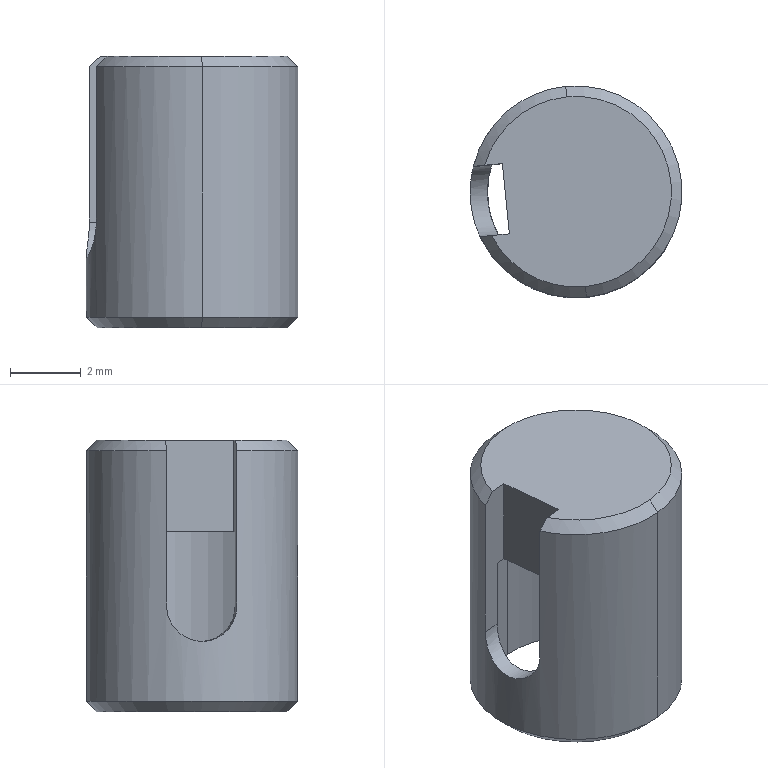Component | SolidWorks | GMotorAxis-2 | 1 solid | 16 faces | box 6 x 6 x 7.7 mm | volume 107 mm3 | plane 6 | cylinder 5 | cone 5 | commonest cylinder face diameters 5.02 x2 6 x2 2 x1
STEP:
#1=CARTESIAN_POINT('',(-0.6367,0.03141,4.504));
#2=VERTEX_POINT('',#1);
#3=CARTESIAN_POINT('',(-0.6174,-0.1653,4.504));
#4=VERTEX_POINT('',#3);
#5=CARTESIAN_POINT('',(-0.6271,-0.06694,4.504));
#6=DIRECTION('',(0.,0.,-1.));
#7=DIRECTION('',(0.09773,-0.9952,0.));
#8=AXIS2_PLACEMENT_3D('',#5,#6,#7);
#9=CIRCLE('',#8,0.09882);
#10=EDGE_CURVE('',#2,#4,#9,.T.);
#11=ORIENTED_EDGE('',*,*,#10,.F.);
#12=CARTESIAN_POINT('',(-0.6367,0.03141,4.303));
#13=VERTEX_POINT('',#12);
#14=CARTESIAN_POINT('',(-0.6367,0.03141,4.504));
#15=DIRECTION('',(0.,0.,-1.));
#16=VECTOR('',#15,39.37);
#17=LINE('',#14,#16);
#18=EDGE_CURVE('',#2,#13,#17,.T.);
#19=ORIENTED_EDGE('',*,*,#18,.T.);
#20=CARTESIAN_POINT('',(-0.6174,-0.1653,4.303));
#21=VERTEX_POINT('',#20);
#22=CARTESIAN_POINT('',(-0.6271,-0.06694,4.303));
#23=DIRECTION('',(0.,0.,1.));
#24=DIRECTION('',(-0.09773,0.9952,0.));
#25=AXIS2_PLACEMENT_3D('',#22,#23,#24);
#26=CIRCLE('',#25,0.09882);
#27=EDGE_CURVE('',#21,#13,#26,.T.);
#28=ORIENTED_EDGE('',*,*,#27,.F.);
#29=CARTESIAN_POINT('',(-0.6174,-0.1653,4.504));
#30=DIRECTION('',(0.,0.,-1.));
#31=VECTOR('',#30,39.37);
#32=LINE('',#29,#31);
#33=EDGE_CURVE('',#4,#21,#32,.T.);
#34=ORIENTED_EDGE('',*,*,#33,.F.);
#35=EDGE_LOOP('',(#11,#19,#28,#34));
#36=FACE_OUTER_BOUND('',#35,.T.);
#37=CARTESIAN_POINT('',(-0.6271,-0.06694,4.504));
#38=DIRECTION('',(0.,0.,-1.));
#39=DIRECTION('',(0.09773,-0.9952,0.));
#40=AXIS2_PLACEMENT_3D('',#37,#38,#39);
#41=CYLINDRICAL_SURFACE('',#40,0.09882);
#42=ADVANCED_FACE('',(#36),#41,.F.);
#43=CARTESIAN_POINT('',(-0.6167,-0.1727,4.303));
#44=VERTEX_POINT('',#43);
#45=CARTESIAN_POINT('',(-0.6375,0.03885,4.303));
#46=VERTEX_POINT('',#45);
#47=CARTESIAN_POINT('',(-0.6271,-0.06694,4.303));
#48=DIRECTION('',(0.,0.,-1.));
#49=DIRECTION('',(-0.09773,0.9952,0.));
#50=AXIS2_PLACEMENT_3D('',#47,#48,#49);
#51=CIRCLE('',#50,0.1063);
#52=EDGE_CURVE('',#44,#46,#51,.T.);
#53=ORIENTED_EDGE('',*,*,#52,.F.);
#54=CARTESIAN_POINT('',(-0.6155,-0.1845,4.315));
#55=VERTEX_POINT('',#54);
#56=CARTESIAN_POINT('',(-0.6155,-0.1845,4.315));
#57=DIRECTION('',(0.06911,-0.7037,0.7071));
#58=VECTOR('',#57,39.37);
#59=LINE('',#56,#58);
#60=EDGE_CURVE('',#44,#55,#59,.T.);
#61=ORIENTED_EDGE('',*,*,#60,.T.);
#62=CARTESIAN_POINT('',(-0.6386,0.05061,4.315));
#63=VERTEX_POINT('',#62);
#64=CARTESIAN_POINT('',(-0.6271,-0.06694,4.315));
#65=DIRECTION('',(0.,0.,1.));
#66=DIRECTION('',(-0.09773,0.9952,0.));
#67=AXIS2_PLACEMENT_3D('',#64,#65,#66);
#68=CIRCLE('',#67,0.1181);
#69=EDGE_CURVE('',#63,#55,#68,.T.);
#70=ORIENTED_EDGE('',*,*,#69,.F.);
#71=CARTESIAN_POINT('',(-0.6386,0.05061,4.315));
#72=DIRECTION('',(-0.06911,0.7037,0.7071));
#73=VECTOR('',#72,39.37);
#74=LINE('',#71,#73);
#75=EDGE_CURVE('',#46,#63,#74,.T.);
#76=ORIENTED_EDGE('',*,*,#75,.F.);
#77=EDGE_LOOP('',(#53,#61,#70,#76));
#78=FACE_OUTER_BOUND('',#77,.T.);
#79=CARTESIAN_POINT('',(-0.6271,-0.06694,4.315));
#80=DIRECTION('',(0.,0.,1.));
#81=DIRECTION('',(-0.09773,0.9952,0.));
#82=AXIS2_PLACEMENT_3D('',#79,#80,#81);
#83=CONICAL_SURFACE('',#82,0.1181,0.7854);
#84=ADVANCED_FACE('',(#78),#83,.T.);
#85=CARTESIAN_POINT('',(-0.6375,0.03885,4.606));
#86=VERTEX_POINT('',#85);
#87=CARTESIAN_POINT('',(-0.7292,-0.03741,4.606));
#88=VERTEX_POINT('',#87);
#89=CARTESIAN_POINT('',(-0.6271,-0.06694,4.606));
#90=DIRECTION('',(0.,0.,1.));
#91=DIRECTION('',(-0.09773,0.9952,0.));
#92=AXIS2_PLACEMENT_3D('',#89,#90,#91);
#93=CIRCLE('',#92,0.1063);
#94=EDGE_CURVE('',#86,#88,#93,.T.);
#95=ORIENTED_EDGE('',*,*,#94,.F.);
#96=CARTESIAN_POINT('',(-0.6386,0.05061,4.594));
#97=VERTEX_POINT('',#96);
#98=CARTESIAN_POINT('',(-0.6375,0.03885,4.606));
#99=DIRECTION('',(-0.06911,0.7037,-0.7071));
#100=VECTOR('',#99,39.37);
#101=LINE('',#98,#100);
#102=EDGE_CURVE('',#86,#97,#101,.T.);
#103=ORIENTED_EDGE('',*,*,#102,.T.);
#104=CARTESIAN_POINT('',(-0.7418,-0.03864,4.594));
#105=VERTEX_POINT('',#104);
#106=CARTESIAN_POINT('',(-0.6271,-0.06694,4.594));
#107=DIRECTION('',(0.,0.,-1.));
#108=DIRECTION('',(-0.09773,0.9952,0.));
#109=AXIS2_PLACEMENT_3D('',#106,#107,#108);
#110=CIRCLE('',#109,0.1181);
#111=EDGE_CURVE('',#105,#97,#110,.T.);
#112=ORIENTED_EDGE('',*,*,#111,.F.);
#113=CARTESIAN_POINT('',(-0.7292,-0.03741,4.606));
#114=CARTESIAN_POINT('',(-0.7334,-0.03782,4.602));
#115=CARTESIAN_POINT('',(-0.7376,-0.03823,4.598));
#116=CARTESIAN_POINT('',(-0.7418,-0.03864,4.594));
#117=B_SPLINE_CURVE_WITH_KNOTS('',3,(#113,#114,#115,#116),.UNSPECIFIED.,.F.,.F.,(4,4),(0.,0.000439),.UNSPECIFIED.);
#118=EDGE_CURVE('',#88,#105,#117,.T.);
#119=ORIENTED_EDGE('',*,*,#118,.F.);
#120=EDGE_LOOP('',(#95,#103,#112,#119));
#121=FACE_OUTER_BOUND('',#120,.T.);
#122=CARTESIAN_POINT('',(-0.6271,-0.06694,4.606));
#123=DIRECTION('',(0.,0.,-1.));
#124=DIRECTION('',(0.09773,-0.9952,0.));
#125=AXIS2_PLACEMENT_3D('',#122,#123,#124);
#126=CONICAL_SURFACE('',#125,0.1063,0.7854);
#127=ADVANCED_FACE('',(#121),#126,.T.);
#128=ORIENTED_EDGE('',*,*,#102,.F.);
#129=CARTESIAN_POINT('',(-0.6167,-0.1727,4.606));
#130=VERTEX_POINT('',#129);
#131=CARTESIAN_POINT('',(-0.6271,-0.06694,4.606));
#132=DIRECTION('',(0.,0.,1.));
#133=DIRECTION('',(-0.09773,0.9952,0.));
#134=AXIS2_PLACEMENT_3D('',#131,#132,#133);
#135=CIRCLE('',#134,0.1063);
#136=EDGE_CURVE('',#130,#86,#135,.T.);
#137=ORIENTED_EDGE('',*,*,#136,.F.);
#138=CARTESIAN_POINT('',(-0.6155,-0.1845,4.594));
#139=VERTEX_POINT('',#138);
#140=CARTESIAN_POINT('',(-0.6167,-0.1727,4.606));
#141=DIRECTION('',(0.06911,-0.7037,-0.7071));
#142=VECTOR('',#141,39.37);
#143=LINE('',#140,#142);
#144=EDGE_CURVE('',#130,#139,#143,.T.);
#145=ORIENTED_EDGE('',*,*,#144,.T.);
#146=CARTESIAN_POINT('',(-0.6271,-0.06694,4.594));
#147=DIRECTION('',(0.,0.,-1.));
#148=DIRECTION('',(-0.09773,0.9952,0.));
#149=AXIS2_PLACEMENT_3D('',#146,#147,#148);
#150=CIRCLE('',#149,0.1181);
#151=EDGE_CURVE('',#97,#139,#150,.T.);
#152=ORIENTED_EDGE('',*,*,#151,.F.);
#153=EDGE_LOOP('',(#128,#137,#145,#152));
#154=FACE_OUTER_BOUND('',#153,.T.);
#155=CARTESIAN_POINT('',(-0.6271,-0.06694,4.606));
#156=DIRECTION('',(0.,0.,-1.));
#157=DIRECTION('',(0.09773,-0.9952,0.));
#158=AXIS2_PLACEMENT_3D('',#155,#156,#157);
#159=CONICAL_SURFACE('',#158,0.1063,0.7854);
#160=ADVANCED_FACE('',(#154),#159,.T.);
#161=ORIENTED_EDGE('',*,*,#111,.T.);
#162=CARTESIAN_POINT('',(-0.6386,0.05061,4.606));
#163=DIRECTION('',(0.,0.,-1.));
#164=VECTOR('',#163,39.37);
#165=LINE('',#162,#164);
#166=EDGE_CURVE('',#97,#63,#165,.T.);
#167=ORIENTED_EDGE('',*,*,#166,.T.);
#168=ORIENTED_EDGE('',*,*,#69,.T.);
#169=CARTESIAN_POINT('',(-0.6155,-0.1845,4.606));
#170=DIRECTION('',(0.,0.,-1.));
#171=VECTOR('',#170,39.37);
#172=LINE('',#169,#171);
#173=EDGE_CURVE('',#139,#55,#172,.T.);
#174=ORIENTED_EDGE('',*,*,#173,.F.);
#175=CARTESIAN_POINT('',(-0.7341,-0.117,4.594));
#176=VERTEX_POINT('',#175);
#177=CARTESIAN_POINT('',(-0.6271,-0.06694,4.594));
#178=DIRECTION('',(0.,0.,-1.));
#179=DIRECTION('',(-0.09773,0.9952,0.));
#180=AXIS2_PLACEMENT_3D('',#177,#178,#179);
#181=CIRCLE('',#180,0.1181);
#182=EDGE_CURVE('',#139,#176,#181,.T.);
#183=ORIENTED_EDGE('',*,*,#182,.T.);
#184=CARTESIAN_POINT('',(-0.7341,-0.117,4.421));
#185=VERTEX_POINT('',#184);
#186=CARTESIAN_POINT('',(-0.7341,-0.117,4.606));
#187=DIRECTION('',(0.,0.,-1.));
#188=VECTOR('',#187,39.37);
#189=LINE('',#186,#188);
#190=EDGE_CURVE('',#176,#185,#189,.T.);
#191=ORIENTED_EDGE('',*,*,#190,.T.);
#192=CARTESIAN_POINT('',(-0.7418,-0.03864,4.421));
#193=VERTEX_POINT('',#192);
#194=CARTESIAN_POINT('',(-0.7418,-0.03864,4.421));
#195=CARTESIAN_POINT('',(-0.7418,-0.03864,4.416));
#196=CARTESIAN_POINT('',(-0.742,-0.03974,4.411));
#197=CARTESIAN_POINT('',(-0.7429,-0.04378,4.401));
#198=CARTESIAN_POINT('',(-0.7435,-0.04678,4.397));
#199=CARTESIAN_POINT('',(-0.7446,-0.05412,4.39));
#200=CARTESIAN_POINT('',(-0.745,-0.05853,4.387));
#201=CARTESIAN_POINT('',(-0.7453,-0.06812,4.383));
#202=CARTESIAN_POINT('',(-0.7451,-0.07327,4.382));
#203=CARTESIAN_POINT('',(-0.7441,-0.08369,4.382));
#204=CARTESIAN_POINT('',(-0.7432,-0.08883,4.383));
#205=CARTESIAN_POINT('',(-0.7411,-0.09812,4.387));
#206=CARTESIAN_POINT('',(-0.7398,-0.1024,4.39));
#207=CARTESIAN_POINT('',(-0.7374,-0.1094,4.397));
#208=CARTESIAN_POINT('',(-0.7362,-0.1122,4.401));
#209=CARTESIAN_POINT('',(-0.7345,-0.116,4.411));
#210=CARTESIAN_POINT('',(-0.7341,-0.117,4.416));
#211=CARTESIAN_POINT('',(-0.7341,-0.117,4.421));
#212=B_SPLINE_CURVE_WITH_KNOTS('',3,(#194,#195,#196,#197,#198,#199,#200,#201,#202,#203,#204,#205,#206,#207,#208,#209,#210,#211),.UNSPECIFIED.,.F.,.F.,(4,2,2,2,2,2,2,2,4),(0.,0.000396,0.0007919,0.001188,0.001584,0.00198,0.002376,0.002772,0.003168),.UNSPECIFIED.);
#213=EDGE_CURVE('',#193,#185,#212,.T.);
#214=ORIENTED_EDGE('',*,*,#213,.F.);
#215=CARTESIAN_POINT('',(-0.7418,-0.03864,4.606));
#216=DIRECTION('',(0.,0.,1.));
#217=VECTOR('',#216,39.37);
#218=LINE('',#215,#217);
#219=EDGE_CURVE('',#193,#105,#218,.T.);
#220=ORIENTED_EDGE('',*,*,#219,.T.);
#221=EDGE_LOOP('',(#161,#167,#168,#174,#183,#191,#214,#220));
#222=FACE_OUTER_BOUND('',#221,.T.);
#223=CARTESIAN_POINT('',(-0.6271,-0.06694,4.606));
#224=DIRECTION('',(0.,0.,-1.));
#225=DIRECTION('',(0.09773,-0.9952,0.));
#226=AXIS2_PLACEMENT_3D('',#223,#224,#225);
#227=CYLINDRICAL_SURFACE('',#226,0.1181);
#228=ADVANCED_FACE('',(#222),#227,.T.);
#229=CARTESIAN_POINT('',(-0.7016,-0.1138,4.504));
#230=VERTEX_POINT('',#229);
#231=CARTESIAN_POINT('',(-0.7093,-0.03545,4.504));
#232=VERTEX_POINT('',#231);
#233=CARTESIAN_POINT('',(-0.7055,-0.07463,4.504));
#234=DIRECTION('',(-0.09773,0.9952,0.));
#235=VECTOR('',#234,39.37);
#236=LINE('',#233,#235);
#237=EDGE_CURVE('',#230,#232,#236,.T.);
#238=ORIENTED_EDGE('',*,*,#237,.F.);
#239=CARTESIAN_POINT('',(-0.7016,-0.1138,4.606));
#240=VERTEX_POINT('',#239);
#241=CARTESIAN_POINT('',(-0.7016,-0.1138,4.382));
#242=DIRECTION('',(-0.,0.,1.));
#243=VECTOR('',#242,39.37);
#244=LINE('',#241,#243);
#245=EDGE_CURVE('',#230,#240,#244,.T.);
#246=ORIENTED_EDGE('',*,*,#245,.T.);
#247=CARTESIAN_POINT('',(-0.7093,-0.03545,4.606));
#248=VERTEX_POINT('',#247);
#249=CARTESIAN_POINT('',(-0.7055,-0.07463,4.606));
#250=DIRECTION('',(-0.09773,0.9952,0.));
#251=VECTOR('',#250,39.37);
#252=LINE('',#249,#251);
#253=EDGE_CURVE('',#240,#248,#252,.T.);
#254=ORIENTED_EDGE('',*,*,#253,.T.);
#255=CARTESIAN_POINT('',(-0.7093,-0.03545,4.382));
#256=DIRECTION('',(0.,-0.,-1.));
#257=VECTOR('',#256,39.37);
#258=LINE('',#255,#257);
#259=EDGE_CURVE('',#248,#232,#258,.T.);
#260=ORIENTED_EDGE('',*,*,#259,.T.);
#261=EDGE_LOOP('',(#238,#246,#254,#260));
#262=FACE_OUTER_BOUND('',#261,.T.);
#263=CARTESIAN_POINT('',(-0.7055,-0.07463,4.303));
#264=DIRECTION('',(0.9952,0.09773,0.));
#265=DIRECTION('',(0.,0.,-1.));
#266=AXIS2_PLACEMENT_3D('',#263,#264,#265);
#267=PLANE('',#266);
#268=ADVANCED_FACE('',(#262),#267,.F.);
#269=CARTESIAN_POINT('',(-0.7134,-0.115,4.421));
#270=VERTEX_POINT('',#269);
#271=CARTESIAN_POINT('',(-0.7016,-0.1138,4.421));
#272=DIRECTION('',(-0.9952,-0.09773,0.));
#273=VECTOR('',#272,39.37);
#274=LINE('',#271,#273);
#275=EDGE_CURVE('',#270,#185,#274,.T.);
#276=ORIENTED_EDGE('',*,*,#275,.F.);
#277=CARTESIAN_POINT('',(-0.7211,-0.03661,4.421));
#278=VERTEX_POINT('',#277);
#279=CARTESIAN_POINT('',(-0.7134,-0.115,4.421));
#280=CARTESIAN_POINT('',(-0.7134,-0.115,4.416));
#281=CARTESIAN_POINT('',(-0.714,-0.114,4.411));
#282=CARTESIAN_POINT('',(-0.716,-0.1102,4.401));
#283=CARTESIAN_POINT('',(-0.7173,-0.1074,4.397));
#284=CARTESIAN_POINT('',(-0.7201,-0.1004,4.39));
#285=CARTESIAN_POINT('',(-0.7216,-0.09623,4.387));
#286=CARTESIAN_POINT('',(-0.724,-0.08696,4.383));
#287=CARTESIAN_POINT('',(-0.7249,-0.08182,4.382));
#288=CARTESIAN_POINT('',(-0.7259,-0.07147,4.382));
#289=CARTESIAN_POINT('',(-0.726,-0.06627,4.383));
#290=CARTESIAN_POINT('',(-0.7255,-0.05656,4.387));
#291=CARTESIAN_POINT('',(-0.7249,-0.05219,4.39));
#292=CARTESIAN_POINT('',(-0.7235,-0.04481,4.397));
#293=CARTESIAN_POINT('',(-0.7227,-0.04181,4.401));
#294=CARTESIAN_POINT('',(-0.7215,-0.03773,4.411));
#295=CARTESIAN_POINT('',(-0.7211,-0.03661,4.416));
#296=CARTESIAN_POINT('',(-0.7211,-0.03661,4.421));
#297=B_SPLINE_CURVE_WITH_KNOTS('',3,(#279,#280,#281,#282,#283,#284,#285,#286,#287,#288,#289,#290,#291,#292,#293,#294,#295,#296),.UNSPECIFIED.,.F.,.F.,(4,2,2,2,2,2,2,2,4),(0.,0.0003948,0.0007895,0.001184,0.001579,0.001974,0.002369,0.002763,0.003158),.UNSPECIFIED.);
#298=EDGE_CURVE('',#270,#278,#297,.T.);
#299=ORIENTED_EDGE('',*,*,#298,.T.);
#300=CARTESIAN_POINT('',(-0.7093,-0.03545,4.421));
#301=DIRECTION('',(0.9952,0.09773,0.));
#302=VECTOR('',#301,39.37);
#303=LINE('',#300,#302);
#304=EDGE_CURVE('',#193,#278,#303,.T.);
#305=ORIENTED_EDGE('',*,*,#304,.F.);
#306=ORIENTED_EDGE('',*,*,#213,.T.);
#307=EDGE_LOOP('',(#276,#299,#305,#306));
#308=FACE_OUTER_BOUND('',#307,.T.);
#309=CARTESIAN_POINT('',(-0.7055,-0.07463,4.421));
#310=DIRECTION('',(-0.9952,-0.09773,0.));
#311=DIRECTION('',(0.,0.,1.));
#312=AXIS2_PLACEMENT_3D('',#309,#310,#311);
#313=CYLINDRICAL_SURFACE('',#312,0.03937);
#314=ADVANCED_FACE('',(#308),#313,.F.);
#315=ORIENTED_EDGE('',*,*,#166,.F.);
#316=ORIENTED_EDGE('',*,*,#151,.T.);
#317=ORIENTED_EDGE('',*,*,#173,.T.);
#318=CARTESIAN_POINT('',(-0.6271,-0.06694,4.315));
#319=DIRECTION('',(0.,0.,1.));
#320=DIRECTION('',(-0.09773,0.9952,0.));
#321=AXIS2_PLACEMENT_3D('',#318,#319,#320);
#322=CIRCLE('',#321,0.1181);
#323=EDGE_CURVE('',#55,#63,#322,.T.);
#324=ORIENTED_EDGE('',*,*,#323,.T.);
#325=EDGE_LOOP('',(#315,#316,#317,#324));
#326=FACE_OUTER_BOUND('',#325,.T.);
#327=CARTESIAN_POINT('',(-0.6271,-0.06694,4.606));
#328=DIRECTION('',(0.,0.,-1.));
#329=DIRECTION('',(0.09773,-0.9952,0.));
#330=AXIS2_PLACEMENT_3D('',#327,#328,#329);
#331=CYLINDRICAL_SURFACE('',#330,0.1181);
#332=ADVANCED_FACE('',(#326),#331,.T.);
#333=CARTESIAN_POINT('',(-0.7215,-0.1158,4.606));
#334=VERTEX_POINT('',#333);
#335=CARTESIAN_POINT('',(-0.6232,-0.1061,4.606));
#336=DIRECTION('',(0.9952,0.09773,0.));
#337=VECTOR('',#336,39.37);
#338=LINE('',#335,#337);
#339=EDGE_CURVE('',#334,#240,#338,.T.);
#340=ORIENTED_EDGE('',*,*,#339,.F.);
#341=CARTESIAN_POINT('',(-0.6271,-0.06694,4.606));
#342=DIRECTION('',(0.,0.,1.));
#343=DIRECTION('',(-0.09773,0.9952,0.));
#344=AXIS2_PLACEMENT_3D('',#341,#342,#343);
#345=CIRCLE('',#344,0.1063);
#346=EDGE_CURVE('',#334,#130,#345,.T.);
#347=ORIENTED_EDGE('',*,*,#346,.T.);
#348=ORIENTED_EDGE('',*,*,#136,.T.);
#349=ORIENTED_EDGE('',*,*,#94,.T.);
#350=CARTESIAN_POINT('',(-0.6309,-0.02775,4.606));
#351=DIRECTION('',(-0.9952,-0.09773,0.));
#352=VECTOR('',#351,39.37);
#353=LINE('',#350,#352);
#354=EDGE_CURVE('',#248,#88,#353,.T.);
#355=ORIENTED_EDGE('',*,*,#354,.F.);
#356=ORIENTED_EDGE('',*,*,#253,.F.);
#357=EDGE_LOOP('',(#340,#347,#348,#349,#355,#356));
#358=FACE_OUTER_BOUND('',#357,.T.);
#359=CARTESIAN_POINT('',(-0.6271,-0.06694,4.606));
#360=DIRECTION('',(0.,0.,1.));
#361=DIRECTION('',(-0.09773,0.9952,0.));
#362=AXIS2_PLACEMENT_3D('',#359,#360,#361);
#363=PLANE('',#362);
#364=ADVANCED_FACE('',(#358),#363,.T.);
#365=ORIENTED_EDGE('',*,*,#27,.T.);
#366=CARTESIAN_POINT('',(-0.6271,-0.06694,4.303));
#367=DIRECTION('',(0.,0.,1.));
#368=DIRECTION('',(-0.09773,0.9952,0.));
#369=AXIS2_PLACEMENT_3D('',#366,#367,#368);
#370=CIRCLE('',#369,0.09882);
#371=EDGE_CURVE('',#13,#21,#370,.T.);
#372=ORIENTED_EDGE('',*,*,#371,.T.);
#373=EDGE_LOOP('',(#365,#372));
#374=FACE_BOUND('',#373,.T.);
#375=CARTESIAN_POINT('',(-0.6271,-0.06694,4.303));
#376=DIRECTION('',(0.,0.,-1.));
#377=DIRECTION('',(-0.09773,0.9952,0.));
#378=AXIS2_PLACEMENT_3D('',#375,#376,#377);
#379=CIRCLE('',#378,0.1063);
#380=EDGE_CURVE('',#46,#44,#379,.T.);
#381=ORIENTED_EDGE('',*,*,#380,.T.);
#382=ORIENTED_EDGE('',*,*,#52,.T.);
#383=EDGE_LOOP('',(#381,#382));
#384=FACE_OUTER_BOUND('',#383,.T.);
#385=CARTESIAN_POINT('',(-0.6271,-0.06694,4.303));
#386=DIRECTION('',(0.,0.,1.));
#387=DIRECTION('',(-0.09773,0.9952,0.));
#388=AXIS2_PLACEMENT_3D('',#385,#386,#387);
#389=PLANE('',#388);
#390=ADVANCED_FACE('',(#374,#384),#389,.F.);
#391=CARTESIAN_POINT('',(-0.7134,-0.115,4.504));
#392=VERTEX_POINT('',#391);
#393=CARTESIAN_POINT('',(-0.7016,-0.1138,4.504));
#394=DIRECTION('',(0.9952,0.09773,0.));
#395=VECTOR('',#394,39.37);
#396=LINE('',#393,#395);
#397=EDGE_CURVE('',#392,#230,#396,.T.);
#398=ORIENTED_EDGE('',*,*,#397,.F.);
#399=CARTESIAN_POINT('',(-0.7134,-0.115,4.504));
#400=DIRECTION('',(0.,0.,-1.));
#401=VECTOR('',#400,39.37);
#402=LINE('',#399,#401);
#403=EDGE_CURVE('',#392,#270,#402,.T.);
#404=ORIENTED_EDGE('',*,*,#403,.T.);
#405=ORIENTED_EDGE('',*,*,#275,.T.);
#406=ORIENTED_EDGE('',*,*,#190,.F.);
#407=CARTESIAN_POINT('',(-0.7341,-0.117,4.594));
#408=CARTESIAN_POINT('',(-0.7299,-0.1166,4.598));
#409=CARTESIAN_POINT('',(-0.7257,-0.1162,4.602));
#410=CARTESIAN_POINT('',(-0.7215,-0.1158,4.606));
#411=B_SPLINE_CURVE_WITH_KNOTS('',3,(#407,#408,#409,#410),.UNSPECIFIED.,.F.,.F.,(4,4),(0.,0.000439),.UNSPECIFIED.);
#412=EDGE_CURVE('',#176,#334,#411,.T.);
#413=ORIENTED_EDGE('',*,*,#412,.T.);
#414=ORIENTED_EDGE('',*,*,#339,.T.);
#415=ORIENTED_EDGE('',*,*,#245,.F.);
#416=EDGE_LOOP('',(#398,#404,#405,#406,#413,#414,#415));
#417=FACE_OUTER_BOUND('',#416,.T.);
#418=CARTESIAN_POINT('',(-0.7016,-0.1138,4.382));
#419=DIRECTION('',(0.09773,-0.9952,0.));
#420=DIRECTION('',(-0.,0.,1.));
#421=AXIS2_PLACEMENT_3D('',#418,#419,#420);
#422=PLANE('',#421);
#423=ADVANCED_FACE('',(#417),#422,.F.);
#424=ORIENTED_EDGE('',*,*,#304,.T.);
#425=CARTESIAN_POINT('',(-0.7211,-0.03661,4.504));
#426=VERTEX_POINT('',#425);
#427=CARTESIAN_POINT('',(-0.7211,-0.03661,4.504));
#428=DIRECTION('',(0.,0.,1.));
#429=VECTOR('',#428,39.37);
#430=LINE('',#427,#429);
#431=EDGE_CURVE('',#278,#426,#430,.T.);
#432=ORIENTED_EDGE('',*,*,#431,.T.);
#433=CARTESIAN_POINT('',(-0.7093,-0.03545,4.504));
#434=DIRECTION('',(-0.9952,-0.09773,0.));
#435=VECTOR('',#434,39.37);
#436=LINE('',#433,#435);
#437=EDGE_CURVE('',#232,#426,#436,.T.);
#438=ORIENTED_EDGE('',*,*,#437,.F.);
#439=ORIENTED_EDGE('',*,*,#259,.F.);
#440=ORIENTED_EDGE('',*,*,#354,.T.);
#441=ORIENTED_EDGE('',*,*,#118,.T.);
#442=ORIENTED_EDGE('',*,*,#219,.F.);
#443=EDGE_LOOP('',(#424,#432,#438,#439,#440,#441,#442));
#444=FACE_OUTER_BOUND('',#443,.T.);
#445=CARTESIAN_POINT('',(-0.7093,-0.03545,4.382));
#446=DIRECTION('',(-0.09773,0.9952,-0.));
#447=DIRECTION('',(0.,-0.,-1.));
#448=AXIS2_PLACEMENT_3D('',#445,#446,#447);
#449=PLANE('',#448);
#450=ADVANCED_FACE('',(#444),#449,.F.);
#451=ORIENTED_EDGE('',*,*,#144,.F.);
#452=ORIENTED_EDGE('',*,*,#346,.F.);
#453=ORIENTED_EDGE('',*,*,#412,.F.);
#454=ORIENTED_EDGE('',*,*,#182,.F.);
#455=EDGE_LOOP('',(#451,#452,#453,#454));
#456=FACE_OUTER_BOUND('',#455,.T.);
#457=CARTESIAN_POINT('',(-0.6271,-0.06694,4.606));
#458=DIRECTION('',(0.,0.,-1.));
#459=DIRECTION('',(0.09773,-0.9952,0.));
#460=AXIS2_PLACEMENT_3D('',#457,#458,#459);
#461=CONICAL_SURFACE('',#460,0.1063,0.7854);
#462=ADVANCED_FACE('',(#456),#461,.T.);
#463=ORIENTED_EDGE('',*,*,#60,.F.);
#464=ORIENTED_EDGE('',*,*,#380,.F.);
#465=ORIENTED_EDGE('',*,*,#75,.T.);
#466=ORIENTED_EDGE('',*,*,#323,.F.);
#467=EDGE_LOOP('',(#463,#464,#465,#466));
#468=FACE_OUTER_BOUND('',#467,.T.);
#469=CARTESIAN_POINT('',(-0.6271,-0.06694,4.315));
#470=DIRECTION('',(0.,0.,1.));
#471=DIRECTION('',(-0.09773,0.9952,0.));
#472=AXIS2_PLACEMENT_3D('',#469,#470,#471);
#473=CONICAL_SURFACE('',#472,0.1181,0.7854);
#474=ADVANCED_FACE('',(#468),#473,.T.);
#475=ORIENTED_EDGE('',*,*,#18,.F.);
#476=CARTESIAN_POINT('',(-0.6271,-0.06694,4.504));
#477=DIRECTION('',(0.,0.,-1.));
#478=DIRECTION('',(0.09773,-0.9952,0.));
#479=AXIS2_PLACEMENT_3D('',#476,#477,#478);
#480=CIRCLE('',#479,0.09882);
#481=EDGE_CURVE('',#426,#2,#480,.T.);
#482=ORIENTED_EDGE('',*,*,#481,.F.);
#483=ORIENTED_EDGE('',*,*,#431,.F.);
#484=ORIENTED_EDGE('',*,*,#298,.F.);
#485=ORIENTED_EDGE('',*,*,#403,.F.);
#486=CARTESIAN_POINT('',(-0.6271,-0.06694,4.504));
#487=DIRECTION('',(0.,0.,-1.));
#488=DIRECTION('',(0.09773,-0.9952,0.));
#489=AXIS2_PLACEMENT_3D('',#486,#487,#488);
#490=CIRCLE('',#489,0.09882);
#491=EDGE_CURVE('',#4,#392,#490,.T.);
#492=ORIENTED_EDGE('',*,*,#491,.F.);
#493=ORIENTED_EDGE('',*,*,#33,.T.);
#494=ORIENTED_EDGE('',*,*,#371,.F.);
#495=EDGE_LOOP('',(#475,#482,#483,#484,#485,#492,#493,#494));
#496=FACE_OUTER_BOUND('',#495,.T.);
#497=CARTESIAN_POINT('',(-0.6271,-0.06694,4.504));
#498=DIRECTION('',(0.,0.,-1.));
#499=DIRECTION('',(0.09773,-0.9952,0.));
#500=AXIS2_PLACEMENT_3D('',#497,#498,#499);
#501=CYLINDRICAL_SURFACE('',#500,0.09882);
#502=ADVANCED_FACE('',(#496),#501,.F.);
#503=ORIENTED_EDGE('',*,*,#397,.T.);
#504=ORIENTED_EDGE('',*,*,#237,.T.);
#505=ORIENTED_EDGE('',*,*,#437,.T.);
#506=ORIENTED_EDGE('',*,*,#481,.T.);
#507=ORIENTED_EDGE('',*,*,#10,.T.);
#508=ORIENTED_EDGE('',*,*,#491,.T.);
#509=EDGE_LOOP('',(#503,#504,#505,#506,#507,#508));
#510=FACE_OUTER_BOUND('',#509,.T.);
#511=CARTESIAN_POINT('',(-0.6271,-0.06694,4.504));
#512=DIRECTION('',(0.,0.,-1.));
#513=DIRECTION('',(0.09773,-0.9952,0.));
#514=AXIS2_PLACEMENT_3D('',#511,#512,#513);
#515=PLANE('',#514);
#516=ADVANCED_FACE('',(#510),#515,.T.);
#517=CLOSED_SHELL('',(#42,#84,#127,#160,#228,#268,#314,#332,#364,#390,#423,#450,#462,#474,#502,#516));
#518=MANIFOLD_SOLID_BREP('',#517);
#519=CARTESIAN_POINT('',(0.,0.,0.));
#520=DIRECTION('',(0.,0.,1.));
#521=DIRECTION('',(1.,0.,0.));
#522=AXIS2_PLACEMENT_3D('',#519,#520,#521);
#523=(LENGTH_UNIT()NAMED_UNIT(*)SI_UNIT($,.METRE.));
#524=LENGTH_MEASURE_WITH_UNIT(LENGTH_MEASURE(0.0254),#523);
#525=DIMENSIONAL_EXPONENTS(1.,0.,0.,0.,0.,0.,0.);
#526=(CONVERSION_BASED_UNIT('',#524)LENGTH_UNIT()NAMED_UNIT(#525));
#527=UNCERTAINTY_MEASURE_WITH_UNIT(LENGTH_MEASURE(0.00001),#526,'','');
#528=(NAMED_UNIT(*)PLANE_ANGLE_UNIT()SI_UNIT($,.RADIAN.));
#529=(NAMED_UNIT(*)SI_UNIT($,.STERADIAN.)SOLID_ANGLE_UNIT());
#530=(GEOMETRIC_REPRESENTATION_CONTEXT(3)GLOBAL_UNCERTAINTY_ASSIGNED_CONTEXT((#527))GLOBAL_UNIT_ASSIGNED_CONTEXT((#526,#528,#529))REPRESENTATION_CONTEXT('',''));
#531=ADVANCED_BREP_SHAPE_REPRESENTATION('',(#518,#522),#530);
#532=COLOUR_RGB('',0.7922,0.8196,0.9333);
#533=FILL_AREA_STYLE_COLOUR('',#532);
#534=FILL_AREA_STYLE('',(#533));
#535=SURFACE_STYLE_FILL_AREA(#534);
#536=SURFACE_SIDE_STYLE('',(#535));
#537=SURFACE_STYLE_USAGE(.BOTH.,#536);
#538=PRESENTATION_STYLE_ASSIGNMENT((#537));
#539=STYLED_ITEM('',(#538),#518);
#540=PRESENTATION_LAYER_ASSIGNMENT('','',(#539));
#541=(LENGTH_UNIT()NAMED_UNIT(*)SI_UNIT($,.METRE.));
#542=LENGTH_MEASURE_WITH_UNIT(LENGTH_MEASURE(0.0254),#541);
#543=DIMENSIONAL_EXPONENTS(1.,0.,0.,0.,0.,0.,0.);
#544=(CONVERSION_BASED_UNIT('',#542)LENGTH_UNIT()NAMED_UNIT(#543));
#545=UNCERTAINTY_MEASURE_WITH_UNIT(LENGTH_MEASURE(0.00001),#544,'','');
#546=(NAMED_UNIT(*)PLANE_ANGLE_UNIT()SI_UNIT($,.RADIAN.));
#547=(NAMED_UNIT(*)SI_UNIT($,.STERADIAN.)SOLID_ANGLE_UNIT());
#548=(GEOMETRIC_REPRESENTATION_CONTEXT(3)GLOBAL_UNCERTAINTY_ASSIGNED_CONTEXT((#545))GLOBAL_UNIT_ASSIGNED_CONTEXT((#544,#546,#547))REPRESENTATION_CONTEXT('',''));
#549=MECHANICAL_DESIGN_GEOMETRIC_PRESENTATION_REPRESENTATION('',(#539),#548);